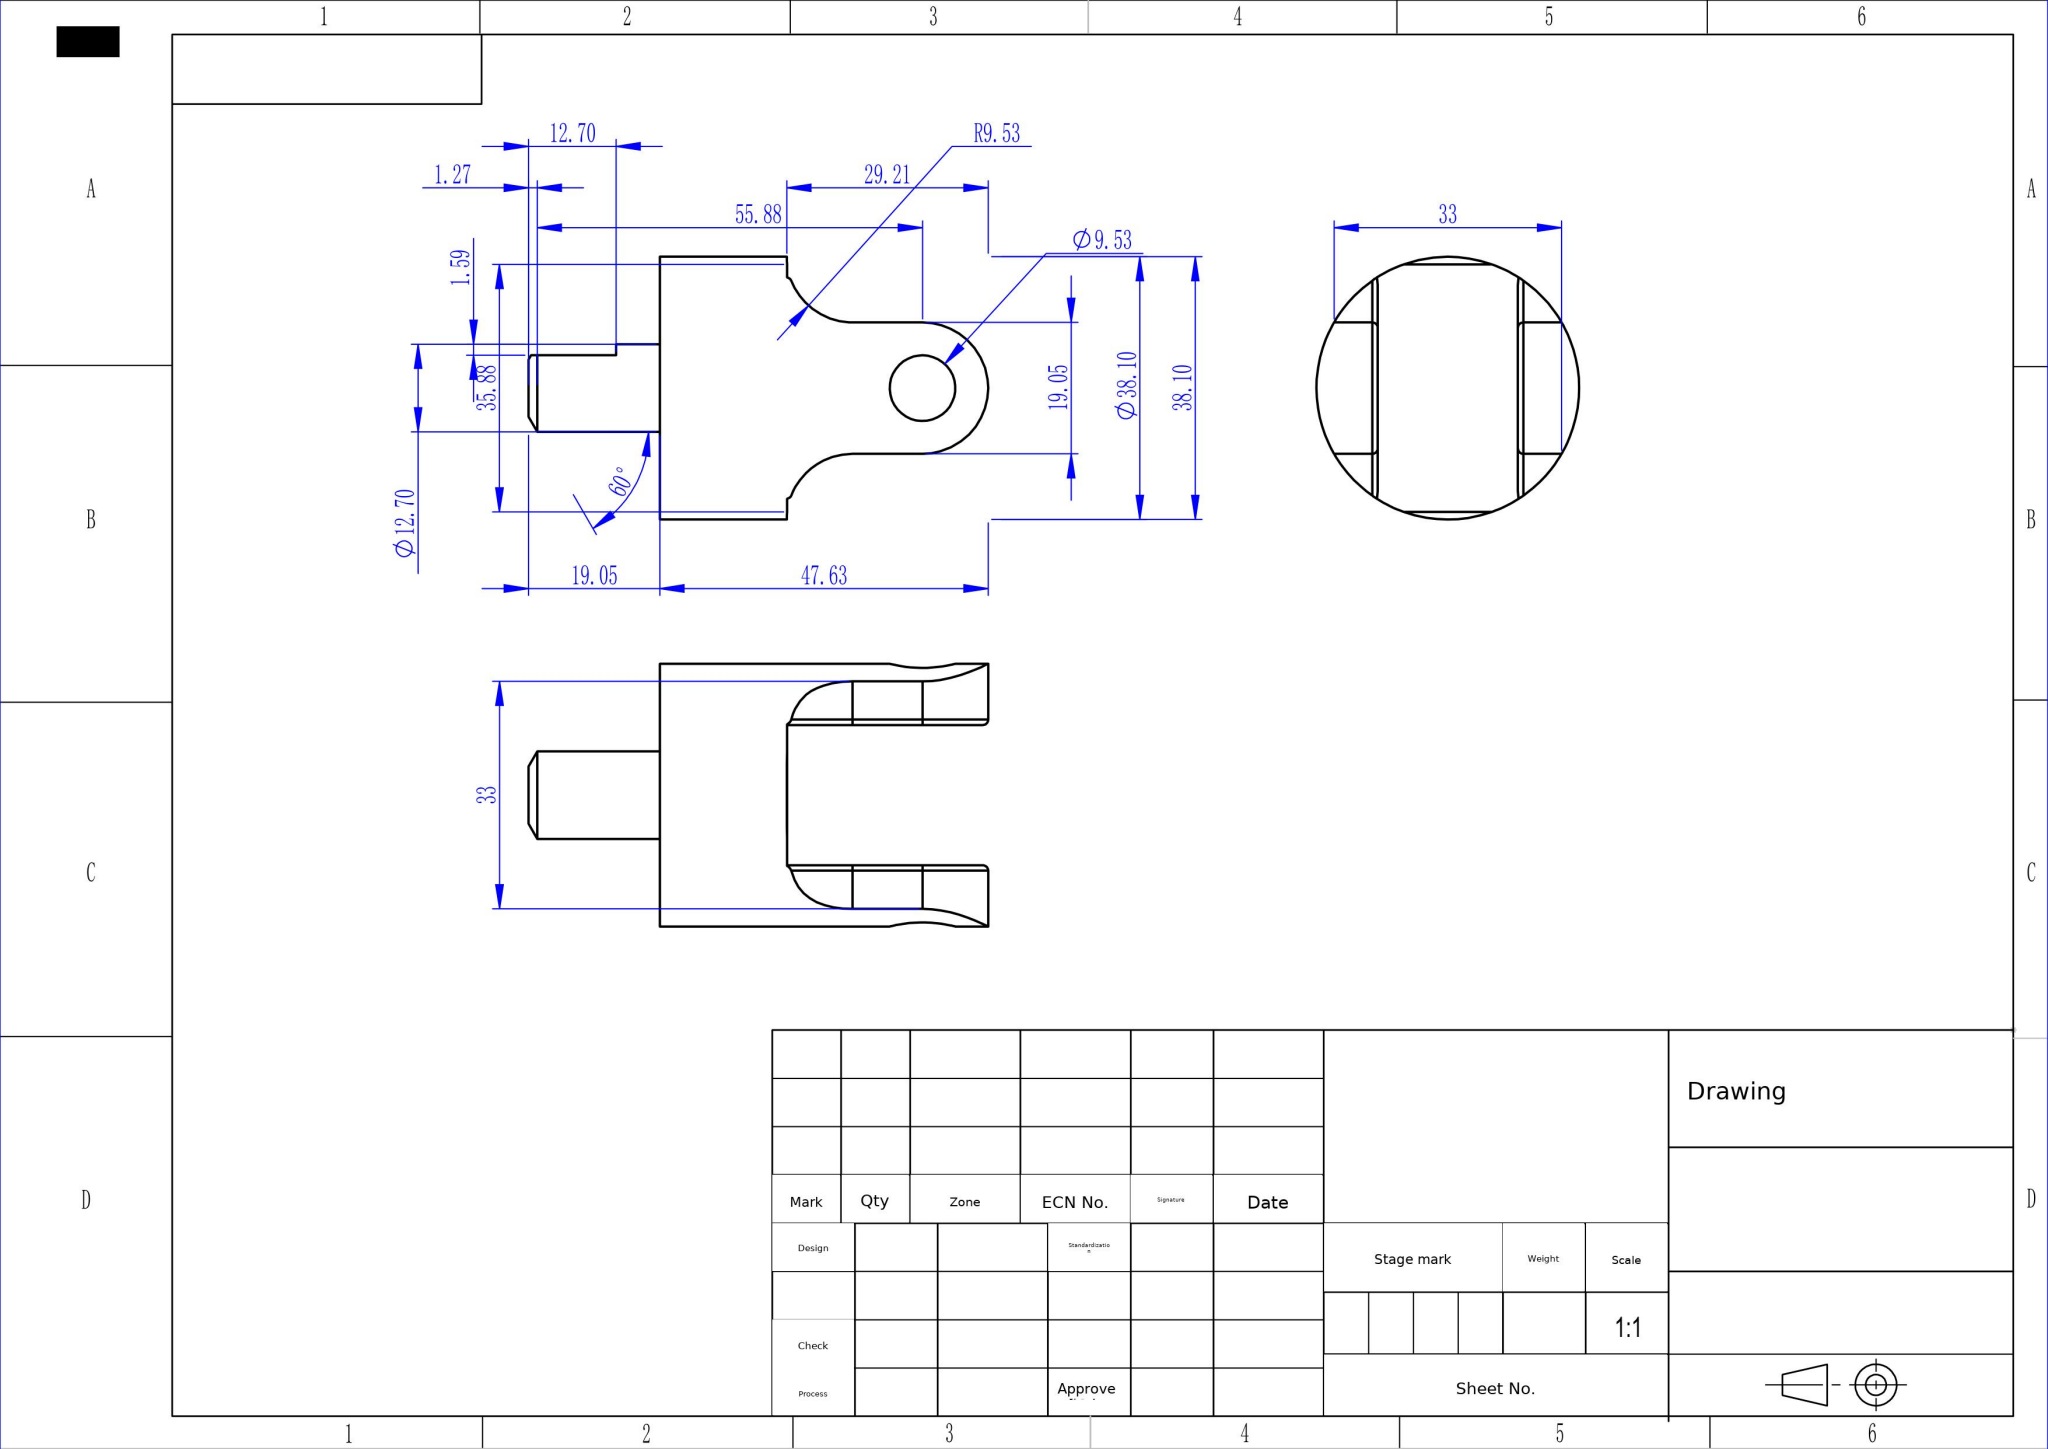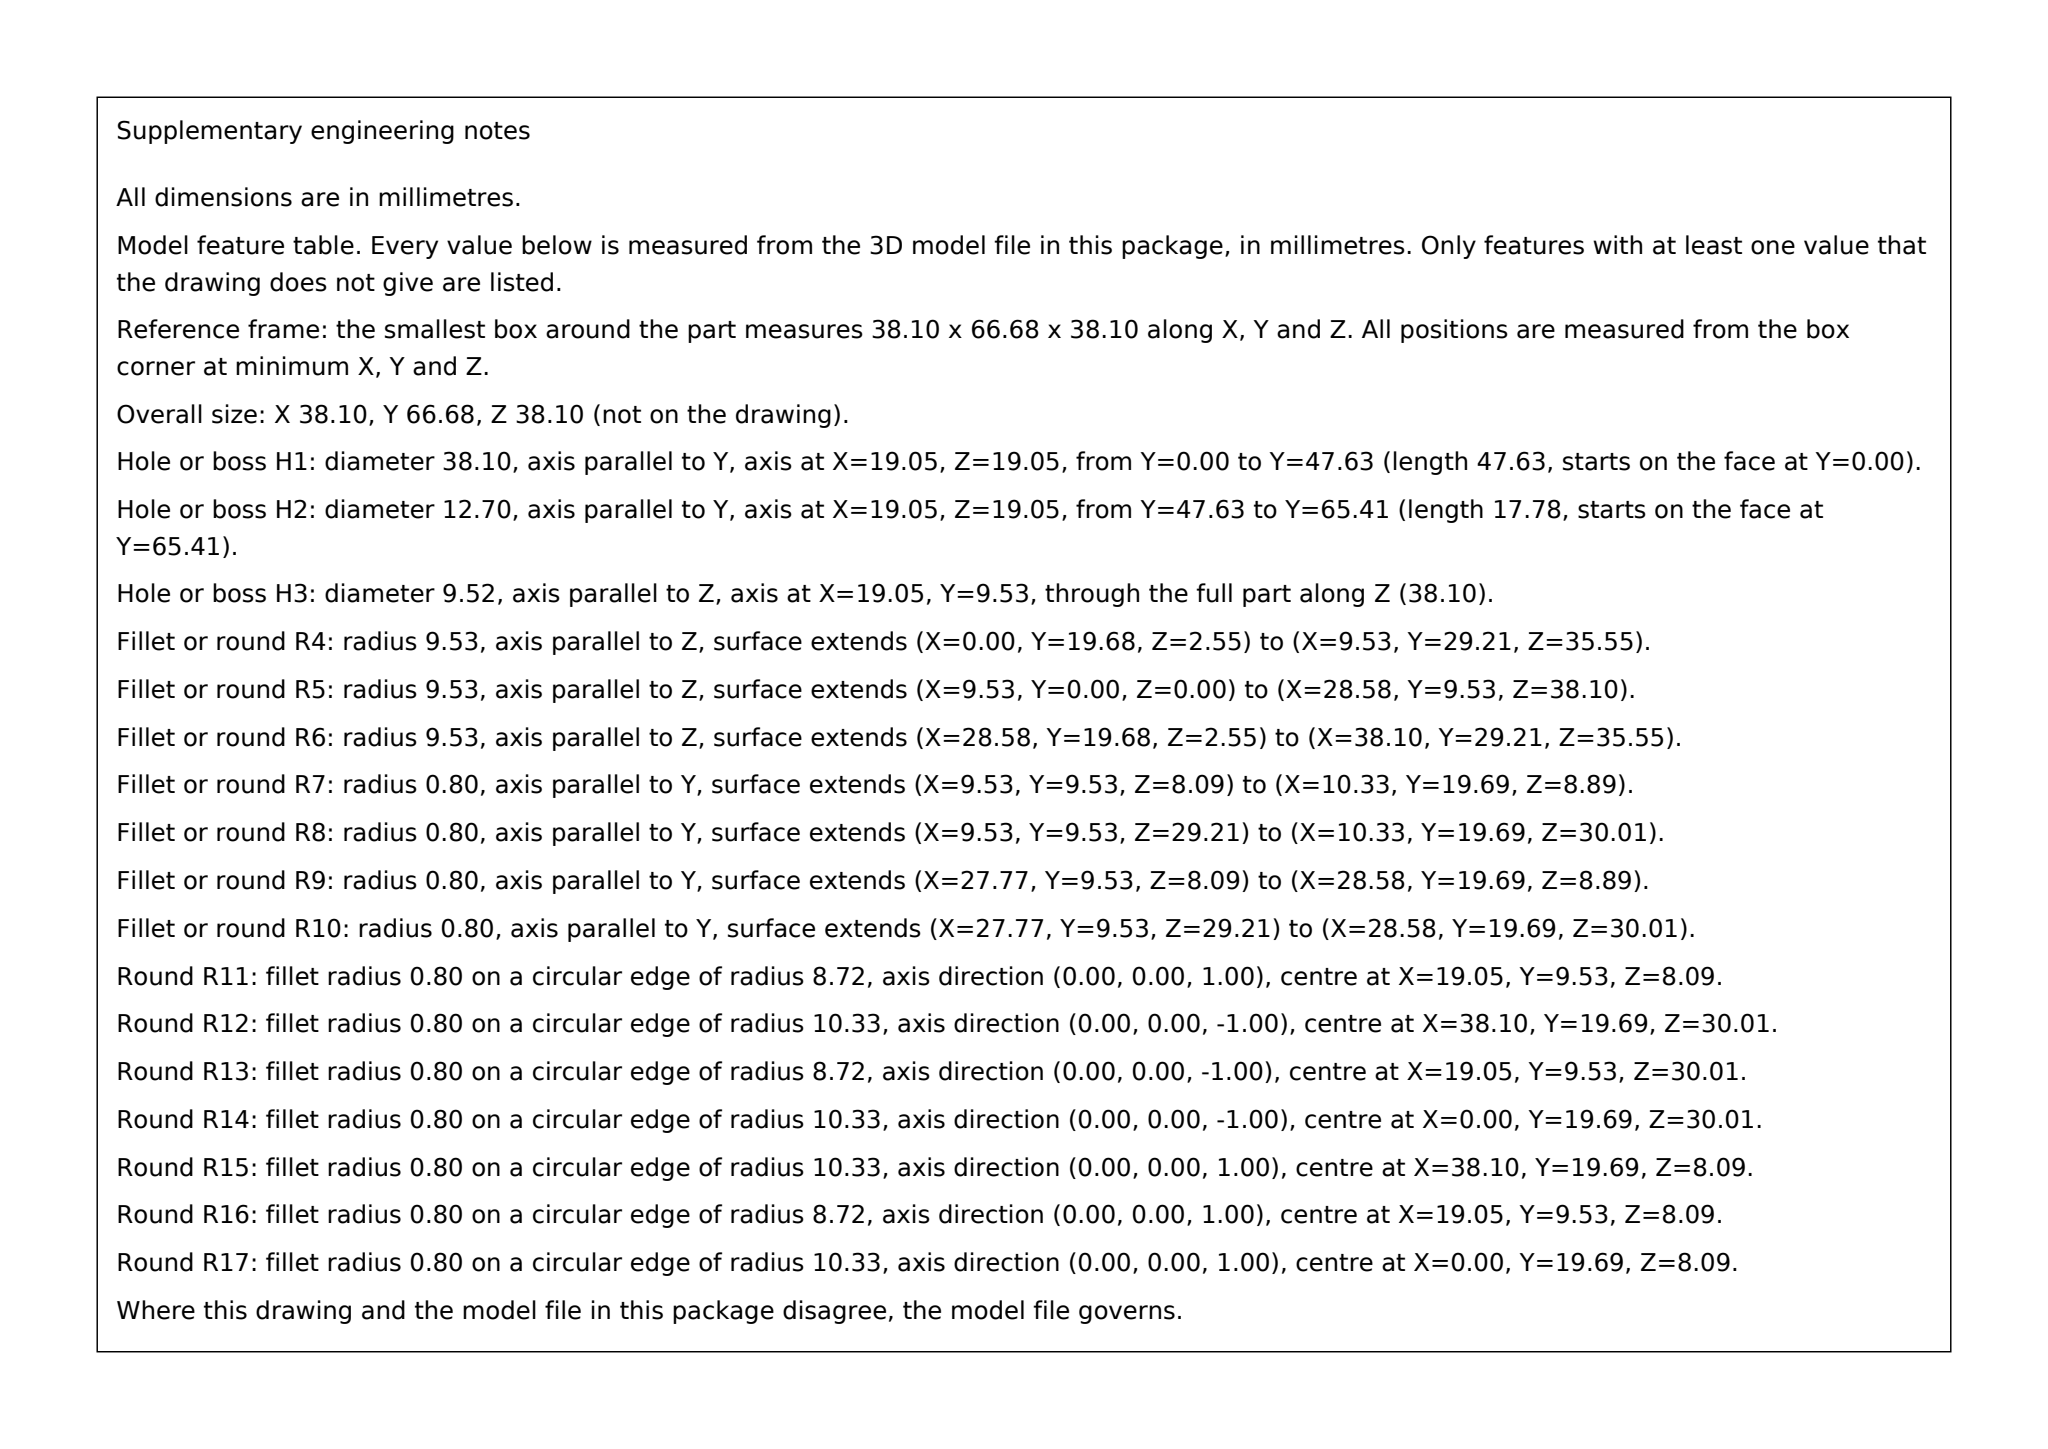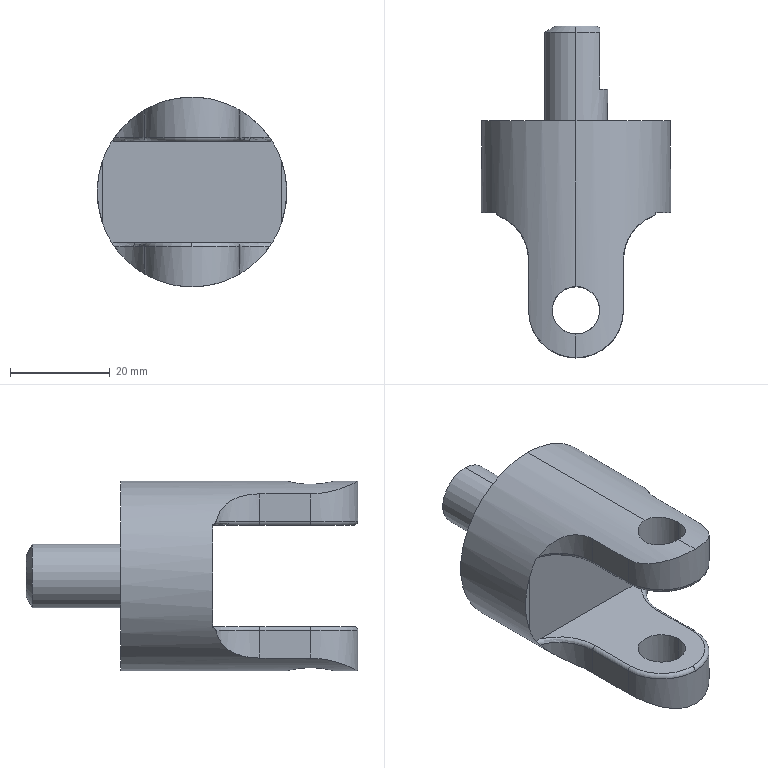Part | SolidWorks | mm | 1 solid | 40 faces | box 38.1 x 66.68 x 38.1 mm | volume 30807 mm3 | cylinder 20 | plane 11 | torus 7 | cone 2 | commonest cylinder face diameters 19.05 x8 9.525 x4 1.6 x4 38.1 x2 12.7 x2